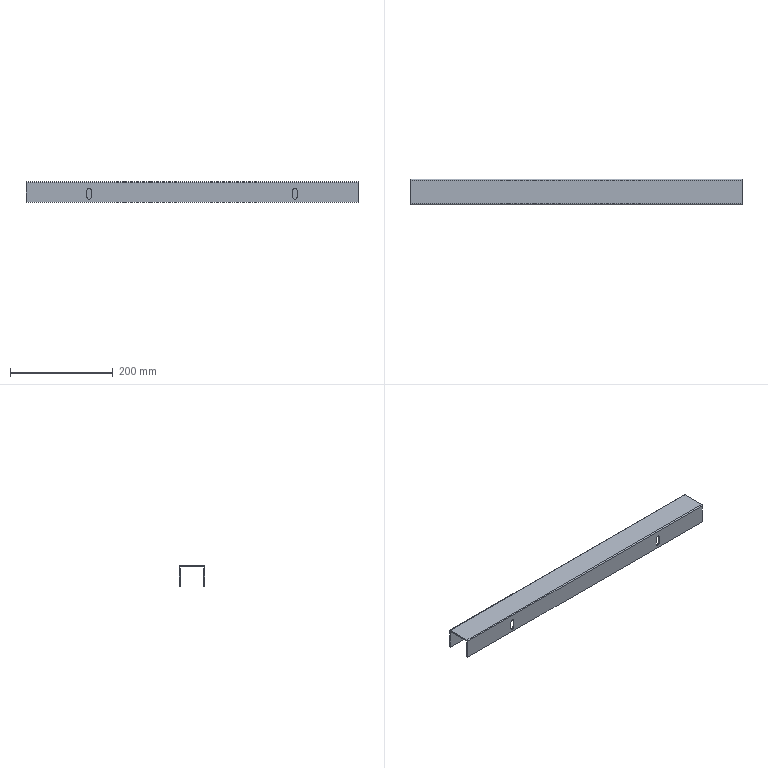Component | SolidWorks | FrameAssembly-1_FrameWeldment-1_FrontBendPlate-1 | 1 solid | 20 faces | box 645 x 50 x 40 mm | volume 199597 mm3 | plane 14 | cylinder 6 | commonest cylinder face diameters 9 x4 4 x2
STEP:
#1=COLOUR_RGB('',0.7922,0.8196,0.9333);
#2=FILL_AREA_STYLE_COLOUR('',#1);
#3=FILL_AREA_STYLE('',(#2));
#4=SURFACE_STYLE_FILL_AREA(#3);
#5=SURFACE_SIDE_STYLE('',(#4));
#6=SURFACE_STYLE_USAGE(.BOTH.,#5);
#7=PRESENTATION_STYLE_ASSIGNMENT((#6));
#8=CARTESIAN_POINT('',(-24.459,-6.068,13.327));
#9=VERTEX_POINT('',#8);
#10=CARTESIAN_POINT('',(0.9352,-6.068,13.327));
#11=VERTEX_POINT('',#10);
#12=CARTESIAN_POINT('',(-24.459,-6.068,13.327));
#13=DIRECTION('',(1.,-0.,-0.));
#14=VECTOR('',#13,39.37);
#15=LINE('',#12,#14);
#16=EDGE_CURVE('',#9,#11,#15,.T.);
#17=ORIENTED_EDGE('',*,*,#16,.T.);
#18=CARTESIAN_POINT('',(0.9352,-6.166,13.327));
#19=VERTEX_POINT('',#18);
#20=CARTESIAN_POINT('',(0.9352,-4.198,13.327));
#21=DIRECTION('',(-0.,-1.,0.));
#22=VECTOR('',#21,39.37);
#23=LINE('',#20,#22);
#24=EDGE_CURVE('',#11,#19,#23,.T.);
#25=ORIENTED_EDGE('',*,*,#24,.T.);
#26=CARTESIAN_POINT('',(-24.459,-6.166,13.327));
#27=VERTEX_POINT('',#26);
#28=CARTESIAN_POINT('',(0.9352,-6.166,13.327));
#29=DIRECTION('',(-1.,0.,0.));
#30=VECTOR('',#29,39.37);
#31=LINE('',#28,#30);
#32=EDGE_CURVE('',#19,#27,#31,.T.);
#33=ORIENTED_EDGE('',*,*,#32,.T.);
#34=CARTESIAN_POINT('',(-24.459,-4.198,13.327));
#35=DIRECTION('',(-0.,-1.,0.));
#36=VECTOR('',#35,39.37);
#37=LINE('',#34,#36);
#38=EDGE_CURVE('',#9,#27,#37,.T.);
#39=ORIENTED_EDGE('',*,*,#38,.F.);
#40=EDGE_LOOP('',(#17,#25,#33,#39));
#41=FACE_OUTER_BOUND('',#40,.T.);
#42=CARTESIAN_POINT('',(0.9352,-4.198,13.327));
#43=DIRECTION('',(-0.,-0.,-1.));
#44=DIRECTION('',(-1.,0.,0.));
#45=AXIS2_PLACEMENT_3D('',#42,#43,#44);
#46=PLANE('',#45);
#47=ADVANCED_FACE('',(#41),#46,.T.);
#48=CARTESIAN_POINT('',(-24.459,-4.198,14.823));
#49=VERTEX_POINT('',#48);
#50=CARTESIAN_POINT('',(-24.459,-4.198,13.327));
#51=VERTEX_POINT('',#50);
#52=CARTESIAN_POINT('',(-24.459,-4.198,14.823));
#53=DIRECTION('',(-0.,-0.,-1.));
#54=VECTOR('',#53,39.37);
#55=LINE('',#52,#54);
#56=EDGE_CURVE('',#49,#51,#55,.T.);
#57=ORIENTED_EDGE('',*,*,#56,.F.);
#58=CARTESIAN_POINT('',(0.9352,-4.198,14.823));
#59=VERTEX_POINT('',#58);
#60=CARTESIAN_POINT('',(0.9352,-4.198,14.823));
#61=DIRECTION('',(-1.,0.,0.));
#62=VECTOR('',#61,39.37);
#63=LINE('',#60,#62);
#64=EDGE_CURVE('',#59,#49,#63,.T.);
#65=ORIENTED_EDGE('',*,*,#64,.F.);
#66=CARTESIAN_POINT('',(0.9352,-4.198,13.327));
#67=VERTEX_POINT('',#66);
#68=CARTESIAN_POINT('',(0.9352,-4.198,14.823));
#69=DIRECTION('',(-0.,-0.,-1.));
#70=VECTOR('',#69,39.37);
#71=LINE('',#68,#70);
#72=EDGE_CURVE('',#59,#67,#71,.T.);
#73=ORIENTED_EDGE('',*,*,#72,.T.);
#74=CARTESIAN_POINT('',(0.9352,-4.198,13.327));
#75=DIRECTION('',(-1.,0.,0.));
#76=VECTOR('',#75,39.37);
#77=LINE('',#74,#76);
#78=EDGE_CURVE('',#67,#51,#77,.T.);
#79=ORIENTED_EDGE('',*,*,#78,.T.);
#80=EDGE_LOOP('',(#57,#65,#73,#79));
#81=FACE_OUTER_BOUND('',#80,.T.);
#82=CARTESIAN_POINT('',(0.9352,-4.198,14.823));
#83=DIRECTION('',(0.,1.,-0.));
#84=DIRECTION('',(1.,-0.,-0.));
#85=AXIS2_PLACEMENT_3D('',#82,#83,#84);
#86=PLANE('',#85);
#87=ADVANCED_FACE('',(#81),#86,.T.);
#88=CARTESIAN_POINT('',(-24.459,-4.277,14.902));
#89=VERTEX_POINT('',#88);
#90=CARTESIAN_POINT('',(-24.459,-4.277,14.823));
#91=DIRECTION('',(-1.,0.,0.));
#92=DIRECTION('',(0.,0.,1.));
#93=AXIS2_PLACEMENT_3D('',#90,#91,#92);
#94=CIRCLE('',#93,0.07874);
#95=EDGE_CURVE('',#89,#49,#94,.T.);
#96=ORIENTED_EDGE('',*,*,#95,.F.);
#97=CARTESIAN_POINT('',(0.9352,-4.277,14.902));
#98=VERTEX_POINT('',#97);
#99=CARTESIAN_POINT('',(0.9352,-4.277,14.902));
#100=DIRECTION('',(-1.,0.,0.));
#101=VECTOR('',#100,39.37);
#102=LINE('',#99,#101);
#103=EDGE_CURVE('',#98,#89,#102,.T.);
#104=ORIENTED_EDGE('',*,*,#103,.F.);
#105=CARTESIAN_POINT('',(0.9352,-4.277,14.823));
#106=DIRECTION('',(-1.,0.,0.));
#107=DIRECTION('',(0.,0.,1.));
#108=AXIS2_PLACEMENT_3D('',#105,#106,#107);
#109=CIRCLE('',#108,0.07874);
#110=EDGE_CURVE('',#98,#59,#109,.T.);
#111=ORIENTED_EDGE('',*,*,#110,.T.);
#112=ORIENTED_EDGE('',*,*,#64,.T.);
#113=EDGE_LOOP('',(#96,#104,#111,#112));
#114=FACE_OUTER_BOUND('',#113,.T.);
#115=CARTESIAN_POINT('',(0.9352,-4.277,14.823));
#116=DIRECTION('',(-1.,0.,0.));
#117=DIRECTION('',(0.,0.,1.));
#118=AXIS2_PLACEMENT_3D('',#115,#116,#117);
#119=CYLINDRICAL_SURFACE('',#118,0.07874);
#120=ADVANCED_FACE('',(#114),#119,.T.);
#121=CARTESIAN_POINT('',(-24.459,-6.088,14.902));
#122=VERTEX_POINT('',#121);
#123=CARTESIAN_POINT('',(-24.459,-6.088,14.902));
#124=DIRECTION('',(0.,1.,0.));
#125=VECTOR('',#124,39.37);
#126=LINE('',#123,#125);
#127=EDGE_CURVE('',#122,#89,#126,.T.);
#128=ORIENTED_EDGE('',*,*,#127,.F.);
#129=CARTESIAN_POINT('',(0.9352,-6.088,14.902));
#130=VERTEX_POINT('',#129);
#131=CARTESIAN_POINT('',(0.9352,-6.088,14.902));
#132=DIRECTION('',(-1.,0.,0.));
#133=VECTOR('',#132,39.37);
#134=LINE('',#131,#133);
#135=EDGE_CURVE('',#130,#122,#134,.T.);
#136=ORIENTED_EDGE('',*,*,#135,.F.);
#137=CARTESIAN_POINT('',(0.9352,-6.088,14.902));
#138=DIRECTION('',(0.,1.,0.));
#139=VECTOR('',#138,39.37);
#140=LINE('',#137,#139);
#141=EDGE_CURVE('',#130,#98,#140,.T.);
#142=ORIENTED_EDGE('',*,*,#141,.T.);
#143=ORIENTED_EDGE('',*,*,#103,.T.);
#144=EDGE_LOOP('',(#128,#136,#142,#143));
#145=FACE_OUTER_BOUND('',#144,.T.);
#146=CARTESIAN_POINT('',(0.9352,-6.088,14.902));
#147=DIRECTION('',(0.,-0.,1.));
#148=DIRECTION('',(-0.,-1.,-0.));
#149=AXIS2_PLACEMENT_3D('',#146,#147,#148);
#150=PLANE('',#149);
#151=ADVANCED_FACE('',(#145),#150,.T.);
#152=CARTESIAN_POINT('',(-24.459,-6.166,14.823));
#153=VERTEX_POINT('',#152);
#154=CARTESIAN_POINT('',(-24.459,-6.088,14.823));
#155=DIRECTION('',(-1.,0.,0.));
#156=DIRECTION('',(0.,0.,1.));
#157=AXIS2_PLACEMENT_3D('',#154,#155,#156);
#158=CIRCLE('',#157,0.07874);
#159=EDGE_CURVE('',#153,#122,#158,.T.);
#160=ORIENTED_EDGE('',*,*,#159,.F.);
#161=CARTESIAN_POINT('',(0.9352,-6.166,14.823));
#162=VERTEX_POINT('',#161);
#163=CARTESIAN_POINT('',(0.9352,-6.166,14.823));
#164=DIRECTION('',(-1.,0.,0.));
#165=VECTOR('',#164,39.37);
#166=LINE('',#163,#165);
#167=EDGE_CURVE('',#162,#153,#166,.T.);
#168=ORIENTED_EDGE('',*,*,#167,.F.);
#169=CARTESIAN_POINT('',(0.9352,-6.088,14.823));
#170=DIRECTION('',(-1.,0.,0.));
#171=DIRECTION('',(0.,0.,1.));
#172=AXIS2_PLACEMENT_3D('',#169,#170,#171);
#173=CIRCLE('',#172,0.07874);
#174=EDGE_CURVE('',#162,#130,#173,.T.);
#175=ORIENTED_EDGE('',*,*,#174,.T.);
#176=ORIENTED_EDGE('',*,*,#135,.T.);
#177=EDGE_LOOP('',(#160,#168,#175,#176));
#178=FACE_OUTER_BOUND('',#177,.T.);
#179=CARTESIAN_POINT('',(0.9352,-6.088,14.823));
#180=DIRECTION('',(-1.,0.,0.));
#181=DIRECTION('',(0.,0.,1.));
#182=AXIS2_PLACEMENT_3D('',#179,#180,#181);
#183=CYLINDRICAL_SURFACE('',#182,0.07874);
#184=ADVANCED_FACE('',(#178),#183,.T.);
#185=CARTESIAN_POINT('',(-19.813,-6.166,13.74));
#186=VERTEX_POINT('',#185);
#187=CARTESIAN_POINT('',(-19.459,-6.166,13.74));
#188=VERTEX_POINT('',#187);
#189=CARTESIAN_POINT('',(-19.636,-6.166,13.74));
#190=DIRECTION('',(-0.,-1.,0.));
#191=DIRECTION('',(-1.,0.,0.));
#192=AXIS2_PLACEMENT_3D('',#189,#190,#191);
#193=CIRCLE('',#192,0.1772);
#194=EDGE_CURVE('',#186,#188,#193,.T.);
#195=ORIENTED_EDGE('',*,*,#194,.F.);
#196=CARTESIAN_POINT('',(-19.813,-6.166,14.213));
#197=VERTEX_POINT('',#196);
#198=CARTESIAN_POINT('',(-19.813,-6.166,14.213));
#199=DIRECTION('',(-0.,-0.,-1.));
#200=VECTOR('',#199,39.37);
#201=LINE('',#198,#200);
#202=EDGE_CURVE('',#197,#186,#201,.T.);
#203=ORIENTED_EDGE('',*,*,#202,.F.);
#204=CARTESIAN_POINT('',(-19.459,-6.166,14.213));
#205=VERTEX_POINT('',#204);
#206=CARTESIAN_POINT('',(-19.636,-6.166,14.213));
#207=DIRECTION('',(-0.,-1.,0.));
#208=DIRECTION('',(-1.,0.,0.));
#209=AXIS2_PLACEMENT_3D('',#206,#207,#208);
#210=CIRCLE('',#209,0.1772);
#211=EDGE_CURVE('',#205,#197,#210,.T.);
#212=ORIENTED_EDGE('',*,*,#211,.F.);
#213=CARTESIAN_POINT('',(-19.459,-6.166,13.74));
#214=DIRECTION('',(0.,0.,1.));
#215=VECTOR('',#214,39.37);
#216=LINE('',#213,#215);
#217=EDGE_CURVE('',#188,#205,#216,.T.);
#218=ORIENTED_EDGE('',*,*,#217,.F.);
#219=EDGE_LOOP('',(#195,#203,#212,#218));
#220=FACE_BOUND('',#219,.T.);
#221=CARTESIAN_POINT('',(-3.71,-6.166,13.74));
#222=VERTEX_POINT('',#221);
#223=CARTESIAN_POINT('',(-4.065,-6.166,13.74));
#224=VERTEX_POINT('',#223);
#225=CARTESIAN_POINT('',(-3.888,-6.166,13.74));
#226=DIRECTION('',(0.,1.,-0.));
#227=DIRECTION('',(1.,0.,0.));
#228=AXIS2_PLACEMENT_3D('',#225,#226,#227);
#229=CIRCLE('',#228,0.1772);
#230=EDGE_CURVE('',#222,#224,#229,.T.);
#231=ORIENTED_EDGE('',*,*,#230,.T.);
#232=CARTESIAN_POINT('',(-4.065,-6.166,14.213));
#233=VERTEX_POINT('',#232);
#234=CARTESIAN_POINT('',(-4.065,-6.166,13.74));
#235=DIRECTION('',(0.,0.,1.));
#236=VECTOR('',#235,39.37);
#237=LINE('',#234,#236);
#238=EDGE_CURVE('',#224,#233,#237,.T.);
#239=ORIENTED_EDGE('',*,*,#238,.T.);
#240=CARTESIAN_POINT('',(-3.71,-6.166,14.213));
#241=VERTEX_POINT('',#240);
#242=CARTESIAN_POINT('',(-3.888,-6.166,14.213));
#243=DIRECTION('',(0.,1.,-0.));
#244=DIRECTION('',(1.,0.,0.));
#245=AXIS2_PLACEMENT_3D('',#242,#243,#244);
#246=CIRCLE('',#245,0.1772);
#247=EDGE_CURVE('',#233,#241,#246,.T.);
#248=ORIENTED_EDGE('',*,*,#247,.T.);
#249=CARTESIAN_POINT('',(-3.71,-6.166,14.213));
#250=DIRECTION('',(-0.,-0.,-1.));
#251=VECTOR('',#250,39.37);
#252=LINE('',#249,#251);
#253=EDGE_CURVE('',#241,#222,#252,.T.);
#254=ORIENTED_EDGE('',*,*,#253,.T.);
#255=EDGE_LOOP('',(#231,#239,#248,#254));
#256=FACE_BOUND('',#255,.T.);
#257=CARTESIAN_POINT('',(-24.459,-6.166,13.327));
#258=DIRECTION('',(0.,0.,1.));
#259=VECTOR('',#258,39.37);
#260=LINE('',#257,#259);
#261=EDGE_CURVE('',#27,#153,#260,.T.);
#262=ORIENTED_EDGE('',*,*,#261,.F.);
#263=ORIENTED_EDGE('',*,*,#32,.F.);
#264=CARTESIAN_POINT('',(0.9352,-6.166,13.327));
#265=DIRECTION('',(0.,0.,1.));
#266=VECTOR('',#265,39.37);
#267=LINE('',#264,#266);
#268=EDGE_CURVE('',#19,#162,#267,.T.);
#269=ORIENTED_EDGE('',*,*,#268,.T.);
#270=ORIENTED_EDGE('',*,*,#167,.T.);
#271=EDGE_LOOP('',(#262,#263,#269,#270));
#272=FACE_OUTER_BOUND('',#271,.T.);
#273=CARTESIAN_POINT('',(0.9352,-6.166,13.327));
#274=DIRECTION('',(-0.,-1.,0.));
#275=DIRECTION('',(-1.,0.,0.));
#276=AXIS2_PLACEMENT_3D('',#273,#274,#275);
#277=PLANE('',#276);
#278=ADVANCED_FACE('',(#220,#256,#272),#277,.T.);
#279=CARTESIAN_POINT('',(-24.459,-4.296,13.327));
#280=VERTEX_POINT('',#279);
#281=CARTESIAN_POINT('',(0.9352,-4.296,13.327));
#282=VERTEX_POINT('',#281);
#283=CARTESIAN_POINT('',(-24.459,-4.296,13.327));
#284=DIRECTION('',(1.,-0.,-0.));
#285=VECTOR('',#284,39.37);
#286=LINE('',#283,#285);
#287=EDGE_CURVE('',#280,#282,#286,.T.);
#288=ORIENTED_EDGE('',*,*,#287,.F.);
#289=CARTESIAN_POINT('',(-24.459,-4.198,13.327));
#290=DIRECTION('',(-0.,-1.,0.));
#291=VECTOR('',#290,39.37);
#292=LINE('',#289,#291);
#293=EDGE_CURVE('',#51,#280,#292,.T.);
#294=ORIENTED_EDGE('',*,*,#293,.F.);
#295=ORIENTED_EDGE('',*,*,#78,.F.);
#296=CARTESIAN_POINT('',(0.9352,-4.198,13.327));
#297=DIRECTION('',(-0.,-1.,0.));
#298=VECTOR('',#297,39.37);
#299=LINE('',#296,#298);
#300=EDGE_CURVE('',#67,#282,#299,.T.);
#301=ORIENTED_EDGE('',*,*,#300,.T.);
#302=EDGE_LOOP('',(#288,#294,#295,#301));
#303=FACE_OUTER_BOUND('',#302,.T.);
#304=CARTESIAN_POINT('',(0.9352,-4.198,13.327));
#305=DIRECTION('',(-0.,-0.,-1.));
#306=DIRECTION('',(-1.,0.,0.));
#307=AXIS2_PLACEMENT_3D('',#304,#305,#306);
#308=PLANE('',#307);
#309=ADVANCED_FACE('',(#303),#308,.T.);
#310=ORIENTED_EDGE('',*,*,#24,.F.);
#311=CARTESIAN_POINT('',(0.9352,-6.068,14.803));
#312=VERTEX_POINT('',#311);
#313=CARTESIAN_POINT('',(0.9352,-6.068,14.803));
#314=DIRECTION('',(-0.,-0.,-1.));
#315=VECTOR('',#314,39.37);
#316=LINE('',#313,#315);
#317=EDGE_CURVE('',#312,#11,#316,.T.);
#318=ORIENTED_EDGE('',*,*,#317,.F.);
#319=CARTESIAN_POINT('',(0.9352,-4.296,14.803));
#320=VERTEX_POINT('',#319);
#321=CARTESIAN_POINT('',(0.9352,-4.296,14.803));
#322=DIRECTION('',(-0.,-1.,0.));
#323=VECTOR('',#322,39.37);
#324=LINE('',#321,#323);
#325=EDGE_CURVE('',#320,#312,#324,.T.);
#326=ORIENTED_EDGE('',*,*,#325,.F.);
#327=CARTESIAN_POINT('',(0.9352,-4.296,13.327));
#328=DIRECTION('',(0.,0.,1.));
#329=VECTOR('',#328,39.37);
#330=LINE('',#327,#329);
#331=EDGE_CURVE('',#282,#320,#330,.T.);
#332=ORIENTED_EDGE('',*,*,#331,.F.);
#333=ORIENTED_EDGE('',*,*,#300,.F.);
#334=ORIENTED_EDGE('',*,*,#72,.F.);
#335=ORIENTED_EDGE('',*,*,#110,.F.);
#336=ORIENTED_EDGE('',*,*,#141,.F.);
#337=ORIENTED_EDGE('',*,*,#174,.F.);
#338=ORIENTED_EDGE('',*,*,#268,.F.);
#339=EDGE_LOOP('',(#310,#318,#326,#332,#333,#334,#335,#336,#337,#338));
#340=FACE_OUTER_BOUND('',#339,.T.);
#341=CARTESIAN_POINT('',(0.9352,-6.088,14.823));
#342=DIRECTION('',(-1.,0.,0.));
#343=DIRECTION('',(0.,0.,1.));
#344=AXIS2_PLACEMENT_3D('',#341,#342,#343);
#345=PLANE('',#344);
#346=ADVANCED_FACE('',(#340),#345,.F.);
#347=CARTESIAN_POINT('',(-24.459,-6.068,14.803));
#348=VERTEX_POINT('',#347);
#349=CARTESIAN_POINT('',(-24.459,-6.068,14.803));
#350=DIRECTION('',(-0.,-0.,-1.));
#351=VECTOR('',#350,39.37);
#352=LINE('',#349,#351);
#353=EDGE_CURVE('',#348,#9,#352,.T.);
#354=ORIENTED_EDGE('',*,*,#353,.T.);
#355=ORIENTED_EDGE('',*,*,#38,.T.);
#356=ORIENTED_EDGE('',*,*,#261,.T.);
#357=ORIENTED_EDGE('',*,*,#159,.T.);
#358=ORIENTED_EDGE('',*,*,#127,.T.);
#359=ORIENTED_EDGE('',*,*,#95,.T.);
#360=ORIENTED_EDGE('',*,*,#56,.T.);
#361=ORIENTED_EDGE('',*,*,#293,.T.);
#362=CARTESIAN_POINT('',(-24.459,-4.296,14.803));
#363=VERTEX_POINT('',#362);
#364=CARTESIAN_POINT('',(-24.459,-4.296,13.327));
#365=DIRECTION('',(0.,0.,1.));
#366=VECTOR('',#365,39.37);
#367=LINE('',#364,#366);
#368=EDGE_CURVE('',#280,#363,#367,.T.);
#369=ORIENTED_EDGE('',*,*,#368,.T.);
#370=CARTESIAN_POINT('',(-24.459,-4.296,14.803));
#371=DIRECTION('',(-0.,-1.,0.));
#372=VECTOR('',#371,39.37);
#373=LINE('',#370,#372);
#374=EDGE_CURVE('',#363,#348,#373,.T.);
#375=ORIENTED_EDGE('',*,*,#374,.T.);
#376=EDGE_LOOP('',(#354,#355,#356,#357,#358,#359,#360,#361,#369,#375));
#377=FACE_OUTER_BOUND('',#376,.T.);
#378=CARTESIAN_POINT('',(-24.459,-6.088,14.823));
#379=DIRECTION('',(-1.,0.,0.));
#380=DIRECTION('',(0.,0.,1.));
#381=AXIS2_PLACEMENT_3D('',#378,#379,#380);
#382=PLANE('',#381);
#383=ADVANCED_FACE('',(#377),#382,.T.);
#384=CARTESIAN_POINT('',(-19.813,-6.068,13.74));
#385=VERTEX_POINT('',#384);
#386=CARTESIAN_POINT('',(-19.813,-6.068,14.213));
#387=VERTEX_POINT('',#386);
#388=CARTESIAN_POINT('',(-19.813,-6.068,14.213));
#389=DIRECTION('',(0.,0.,1.));
#390=VECTOR('',#389,39.37);
#391=LINE('',#388,#390);
#392=EDGE_CURVE('',#385,#387,#391,.T.);
#393=ORIENTED_EDGE('',*,*,#392,.F.);
#394=CARTESIAN_POINT('',(-19.459,-6.068,13.74));
#395=VERTEX_POINT('',#394);
#396=CARTESIAN_POINT('',(-19.636,-6.068,13.74));
#397=DIRECTION('',(0.,1.,-0.));
#398=DIRECTION('',(-1.,0.,0.));
#399=AXIS2_PLACEMENT_3D('',#396,#397,#398);
#400=CIRCLE('',#399,0.1772);
#401=EDGE_CURVE('',#395,#385,#400,.T.);
#402=ORIENTED_EDGE('',*,*,#401,.F.);
#403=CARTESIAN_POINT('',(-19.459,-6.068,14.213));
#404=VERTEX_POINT('',#403);
#405=CARTESIAN_POINT('',(-19.459,-6.068,13.74));
#406=DIRECTION('',(-0.,-0.,-1.));
#407=VECTOR('',#406,39.37);
#408=LINE('',#405,#407);
#409=EDGE_CURVE('',#404,#395,#408,.T.);
#410=ORIENTED_EDGE('',*,*,#409,.F.);
#411=CARTESIAN_POINT('',(-19.636,-6.068,14.213));
#412=DIRECTION('',(0.,1.,-0.));
#413=DIRECTION('',(-1.,0.,0.));
#414=AXIS2_PLACEMENT_3D('',#411,#412,#413);
#415=CIRCLE('',#414,0.1772);
#416=EDGE_CURVE('',#387,#404,#415,.T.);
#417=ORIENTED_EDGE('',*,*,#416,.F.);
#418=EDGE_LOOP('',(#393,#402,#410,#417));
#419=FACE_BOUND('',#418,.T.);
#420=CARTESIAN_POINT('',(-4.065,-6.068,13.74));
#421=VERTEX_POINT('',#420);
#422=CARTESIAN_POINT('',(-4.065,-6.068,14.213));
#423=VERTEX_POINT('',#422);
#424=CARTESIAN_POINT('',(-4.065,-6.068,13.74));
#425=DIRECTION('',(0.,0.,1.));
#426=VECTOR('',#425,39.37);
#427=LINE('',#424,#426);
#428=EDGE_CURVE('',#421,#423,#427,.T.);
#429=ORIENTED_EDGE('',*,*,#428,.F.);
#430=CARTESIAN_POINT('',(-3.71,-6.068,13.74));
#431=VERTEX_POINT('',#430);
#432=CARTESIAN_POINT('',(-3.888,-6.068,13.74));
#433=DIRECTION('',(0.,1.,-0.));
#434=DIRECTION('',(1.,0.,0.));
#435=AXIS2_PLACEMENT_3D('',#432,#433,#434);
#436=CIRCLE('',#435,0.1772);
#437=EDGE_CURVE('',#431,#421,#436,.T.);
#438=ORIENTED_EDGE('',*,*,#437,.F.);
#439=CARTESIAN_POINT('',(-3.71,-6.068,14.213));
#440=VERTEX_POINT('',#439);
#441=CARTESIAN_POINT('',(-3.71,-6.068,14.213));
#442=DIRECTION('',(-0.,-0.,-1.));
#443=VECTOR('',#442,39.37);
#444=LINE('',#441,#443);
#445=EDGE_CURVE('',#440,#431,#444,.T.);
#446=ORIENTED_EDGE('',*,*,#445,.F.);
#447=CARTESIAN_POINT('',(-3.888,-6.068,14.213));
#448=DIRECTION('',(0.,1.,-0.));
#449=DIRECTION('',(1.,0.,0.));
#450=AXIS2_PLACEMENT_3D('',#447,#448,#449);
#451=CIRCLE('',#450,0.1772);
#452=EDGE_CURVE('',#423,#440,#451,.T.);
#453=ORIENTED_EDGE('',*,*,#452,.F.);
#454=EDGE_LOOP('',(#429,#438,#446,#453));
#455=FACE_BOUND('',#454,.T.);
#456=ORIENTED_EDGE('',*,*,#317,.T.);
#457=ORIENTED_EDGE('',*,*,#16,.F.);
#458=ORIENTED_EDGE('',*,*,#353,.F.);
#459=CARTESIAN_POINT('',(-24.459,-6.068,14.803));
#460=DIRECTION('',(1.,-0.,-0.));
#461=VECTOR('',#460,39.37);
#462=LINE('',#459,#461);
#463=EDGE_CURVE('',#348,#312,#462,.T.);
#464=ORIENTED_EDGE('',*,*,#463,.T.);
#465=EDGE_LOOP('',(#456,#457,#458,#464));
#466=FACE_OUTER_BOUND('',#465,.T.);
#467=CARTESIAN_POINT('',(-24.459,-6.068,14.803));
#468=DIRECTION('',(-0.,-1.,0.));
#469=DIRECTION('',(-1.,0.,0.));
#470=AXIS2_PLACEMENT_3D('',#467,#468,#469);
#471=PLANE('',#470);
#472=ADVANCED_FACE('',(#419,#455,#466),#471,.F.);
#473=ORIENTED_EDGE('',*,*,#325,.T.);
#474=ORIENTED_EDGE('',*,*,#463,.F.);
#475=ORIENTED_EDGE('',*,*,#374,.F.);
#476=CARTESIAN_POINT('',(-24.459,-4.296,14.803));
#477=DIRECTION('',(1.,-0.,-0.));
#478=VECTOR('',#477,39.37);
#479=LINE('',#476,#478);
#480=EDGE_CURVE('',#363,#320,#479,.T.);
#481=ORIENTED_EDGE('',*,*,#480,.T.);
#482=EDGE_LOOP('',(#473,#474,#475,#481));
#483=FACE_OUTER_BOUND('',#482,.T.);
#484=CARTESIAN_POINT('',(-24.459,-4.296,14.803));
#485=DIRECTION('',(0.,0.,1.));
#486=DIRECTION('',(1.,-0.,-0.));
#487=AXIS2_PLACEMENT_3D('',#484,#485,#486);
#488=PLANE('',#487);
#489=ADVANCED_FACE('',(#483),#488,.F.);
#490=ORIENTED_EDGE('',*,*,#331,.T.);
#491=ORIENTED_EDGE('',*,*,#480,.F.);
#492=ORIENTED_EDGE('',*,*,#368,.F.);
#493=ORIENTED_EDGE('',*,*,#287,.T.);
#494=EDGE_LOOP('',(#490,#491,#492,#493));
#495=FACE_OUTER_BOUND('',#494,.T.);
#496=CARTESIAN_POINT('',(-24.459,-4.296,13.327));
#497=DIRECTION('',(0.,1.,-0.));
#498=DIRECTION('',(1.,-0.,-0.));
#499=AXIS2_PLACEMENT_3D('',#496,#497,#498);
#500=PLANE('',#499);
#501=ADVANCED_FACE('',(#495),#500,.F.);
#502=ORIENTED_EDGE('',*,*,#437,.T.);
#503=CARTESIAN_POINT('',(-4.065,-6.166,13.74));
#504=DIRECTION('',(0.,1.,-0.));
#505=VECTOR('',#504,39.37);
#506=LINE('',#503,#505);
#507=EDGE_CURVE('',#224,#421,#506,.T.);
#508=ORIENTED_EDGE('',*,*,#507,.F.);
#509=ORIENTED_EDGE('',*,*,#230,.F.);
#510=CARTESIAN_POINT('',(-3.71,-6.166,13.74));
#511=DIRECTION('',(0.,1.,-0.));
#512=VECTOR('',#511,39.37);
#513=LINE('',#510,#512);
#514=EDGE_CURVE('',#222,#431,#513,.T.);
#515=ORIENTED_EDGE('',*,*,#514,.T.);
#516=EDGE_LOOP('',(#502,#508,#509,#515));
#517=FACE_OUTER_BOUND('',#516,.T.);
#518=CARTESIAN_POINT('',(-3.888,-6.166,13.74));
#519=DIRECTION('',(0.,1.,-0.));
#520=DIRECTION('',(1.,0.,0.));
#521=AXIS2_PLACEMENT_3D('',#518,#519,#520);
#522=CYLINDRICAL_SURFACE('',#521,0.1772);
#523=ADVANCED_FACE('',(#517),#522,.F.);
#524=ORIENTED_EDGE('',*,*,#445,.T.);
#525=ORIENTED_EDGE('',*,*,#514,.F.);
#526=ORIENTED_EDGE('',*,*,#253,.F.);
#527=CARTESIAN_POINT('',(-3.71,-6.166,14.213));
#528=DIRECTION('',(0.,1.,-0.));
#529=VECTOR('',#528,39.37);
#530=LINE('',#527,#529);
#531=EDGE_CURVE('',#241,#440,#530,.T.);
#532=ORIENTED_EDGE('',*,*,#531,.T.);
#533=EDGE_LOOP('',(#524,#525,#526,#532));
#534=FACE_OUTER_BOUND('',#533,.T.);
#535=CARTESIAN_POINT('',(-3.71,-6.166,14.213));
#536=DIRECTION('',(1.,-0.,-0.));
#537=DIRECTION('',(-0.,-0.,-1.));
#538=AXIS2_PLACEMENT_3D('',#535,#536,#537);
#539=PLANE('',#538);
#540=ADVANCED_FACE('',(#534),#539,.F.);
#541=ORIENTED_EDGE('',*,*,#452,.T.);
#542=ORIENTED_EDGE('',*,*,#531,.F.);
#543=ORIENTED_EDGE('',*,*,#247,.F.);
#544=CARTESIAN_POINT('',(-4.065,-6.166,14.213));
#545=DIRECTION('',(0.,1.,-0.));
#546=VECTOR('',#545,39.37);
#547=LINE('',#544,#546);
#548=EDGE_CURVE('',#233,#423,#547,.T.);
#549=ORIENTED_EDGE('',*,*,#548,.T.);
#550=EDGE_LOOP('',(#541,#542,#543,#549));
#551=FACE_OUTER_BOUND('',#550,.T.);
#552=CARTESIAN_POINT('',(-3.888,-6.166,14.213));
#553=DIRECTION('',(0.,1.,-0.));
#554=DIRECTION('',(1.,0.,0.));
#555=AXIS2_PLACEMENT_3D('',#552,#553,#554);
#556=CYLINDRICAL_SURFACE('',#555,0.1772);
#557=ADVANCED_FACE('',(#551),#556,.F.);
#558=ORIENTED_EDGE('',*,*,#428,.T.);
#559=ORIENTED_EDGE('',*,*,#548,.F.);
#560=ORIENTED_EDGE('',*,*,#238,.F.);
#561=ORIENTED_EDGE('',*,*,#507,.T.);
#562=EDGE_LOOP('',(#558,#559,#560,#561));
#563=FACE_OUTER_BOUND('',#562,.T.);
#564=CARTESIAN_POINT('',(-4.065,-6.166,13.74));
#565=DIRECTION('',(-1.,0.,0.));
#566=DIRECTION('',(0.,0.,1.));
#567=AXIS2_PLACEMENT_3D('',#564,#565,#566);
#568=PLANE('',#567);
#569=ADVANCED_FACE('',(#563),#568,.F.);
#570=ORIENTED_EDGE('',*,*,#401,.T.);
#571=CARTESIAN_POINT('',(-19.813,-4.198,13.74));
#572=DIRECTION('',(-0.,-1.,0.));
#573=VECTOR('',#572,39.37);
#574=LINE('',#571,#573);
#575=EDGE_CURVE('',#385,#186,#574,.T.);
#576=ORIENTED_EDGE('',*,*,#575,.T.);
#577=ORIENTED_EDGE('',*,*,#194,.T.);
#578=CARTESIAN_POINT('',(-19.459,-4.198,13.74));
#579=DIRECTION('',(-0.,-1.,0.));
#580=VECTOR('',#579,39.37);
#581=LINE('',#578,#580);
#582=EDGE_CURVE('',#395,#188,#581,.T.);
#583=ORIENTED_EDGE('',*,*,#582,.F.);
#584=EDGE_LOOP('',(#570,#576,#577,#583));
#585=FACE_OUTER_BOUND('',#584,.T.);
#586=CARTESIAN_POINT('',(-19.636,-4.198,13.74));
#587=DIRECTION('',(-0.,-1.,0.));
#588=DIRECTION('',(-1.,0.,0.));
#589=AXIS2_PLACEMENT_3D('',#586,#587,#588);
#590=CYLINDRICAL_SURFACE('',#589,0.1772);
#591=ADVANCED_FACE('',(#585),#590,.F.);
#592=ORIENTED_EDGE('',*,*,#392,.T.);
#593=CARTESIAN_POINT('',(-19.813,-4.198,14.213));
#594=DIRECTION('',(-0.,-1.,0.));
#595=VECTOR('',#594,39.37);
#596=LINE('',#593,#595);
#597=EDGE_CURVE('',#387,#197,#596,.T.);
#598=ORIENTED_EDGE('',*,*,#597,.T.);
#599=ORIENTED_EDGE('',*,*,#202,.T.);
#600=ORIENTED_EDGE('',*,*,#575,.F.);
#601=EDGE_LOOP('',(#592,#598,#599,#600));
#602=FACE_OUTER_BOUND('',#601,.T.);
#603=CARTESIAN_POINT('',(-19.813,-4.198,14.213));
#604=DIRECTION('',(-1.,0.,0.));
#605=DIRECTION('',(0.,0.,1.));
#606=AXIS2_PLACEMENT_3D('',#603,#604,#605);
#607=PLANE('',#606);
#608=ADVANCED_FACE('',(#602),#607,.F.);
#609=ORIENTED_EDGE('',*,*,#416,.T.);
#610=CARTESIAN_POINT('',(-19.459,-4.198,14.213));
#611=DIRECTION('',(-0.,-1.,0.));
#612=VECTOR('',#611,39.37);
#613=LINE('',#610,#612);
#614=EDGE_CURVE('',#404,#205,#613,.T.);
#615=ORIENTED_EDGE('',*,*,#614,.T.);
#616=ORIENTED_EDGE('',*,*,#211,.T.);
#617=ORIENTED_EDGE('',*,*,#597,.F.);
#618=EDGE_LOOP('',(#609,#615,#616,#617));
#619=FACE_OUTER_BOUND('',#618,.T.);
#620=CARTESIAN_POINT('',(-19.636,-4.198,14.213));
#621=DIRECTION('',(-0.,-1.,0.));
#622=DIRECTION('',(-1.,0.,0.));
#623=AXIS2_PLACEMENT_3D('',#620,#621,#622);
#624=CYLINDRICAL_SURFACE('',#623,0.1772);
#625=ADVANCED_FACE('',(#619),#624,.F.);
#626=ORIENTED_EDGE('',*,*,#409,.T.);
#627=ORIENTED_EDGE('',*,*,#582,.T.);
#628=ORIENTED_EDGE('',*,*,#217,.T.);
#629=ORIENTED_EDGE('',*,*,#614,.F.);
#630=EDGE_LOOP('',(#626,#627,#628,#629));
#631=FACE_OUTER_BOUND('',#630,.T.);
#632=CARTESIAN_POINT('',(-19.459,-4.198,13.74));
#633=DIRECTION('',(1.,-0.,-0.));
#634=DIRECTION('',(-0.,-0.,-1.));
#635=AXIS2_PLACEMENT_3D('',#632,#633,#634);
#636=PLANE('',#635);
#637=ADVANCED_FACE('',(#631),#636,.F.);
#638=CLOSED_SHELL('',(#47,#87,#120,#151,#184,#278,#309,#346,#383,#472,#489,#501,#523,#540,#557,#569,#591,#608,#625,#637));
#639=MANIFOLD_SOLID_BREP('',#638);
#640=STYLED_ITEM('',(#7),#639);
#641=(LENGTH_UNIT()NAMED_UNIT(*)SI_UNIT($,.METRE.));
#642=LENGTH_MEASURE_WITH_UNIT(LENGTH_MEASURE(0.0254),#641);
#643=DIMENSIONAL_EXPONENTS(1.,0.,0.,0.,0.,0.,0.);
#644=(CONVERSION_BASED_UNIT('',#642)LENGTH_UNIT()NAMED_UNIT(#643));
#645=UNCERTAINTY_MEASURE_WITH_UNIT(LENGTH_MEASURE(0.00001),#644,'','');
#646=(NAMED_UNIT(*)PLANE_ANGLE_UNIT()SI_UNIT($,.RADIAN.));
#647=(NAMED_UNIT(*)SI_UNIT($,.STERADIAN.)SOLID_ANGLE_UNIT());
#648=(GEOMETRIC_REPRESENTATION_CONTEXT(3)GLOBAL_UNCERTAINTY_ASSIGNED_CONTEXT((#645))GLOBAL_UNIT_ASSIGNED_CONTEXT((#644,#646,#647))REPRESENTATION_CONTEXT('',''));
#649=MECHANICAL_DESIGN_GEOMETRIC_PRESENTATION_REPRESENTATION('',(#640),#648);
#650=PRESENTATION_LAYER_ASSIGNMENT('','',(#640));
#651=CARTESIAN_POINT('',(0.,0.,0.));
#652=DIRECTION('',(0.,0.,1.));
#653=DIRECTION('',(1.,0.,0.));
#654=AXIS2_PLACEMENT_3D('',#651,#652,#653);
#655=(LENGTH_UNIT()NAMED_UNIT(*)SI_UNIT($,.METRE.));
#656=LENGTH_MEASURE_WITH_UNIT(LENGTH_MEASURE(0.0254),#655);
#657=DIMENSIONAL_EXPONENTS(1.,0.,0.,0.,0.,0.,0.);
#658=(CONVERSION_BASED_UNIT('',#656)LENGTH_UNIT()NAMED_UNIT(#657));
#659=UNCERTAINTY_MEASURE_WITH_UNIT(LENGTH_MEASURE(0.00001),#658,'','');
#660=(NAMED_UNIT(*)PLANE_ANGLE_UNIT()SI_UNIT($,.RADIAN.));
#661=(NAMED_UNIT(*)SI_UNIT($,.STERADIAN.)SOLID_ANGLE_UNIT());
#662=(GEOMETRIC_REPRESENTATION_CONTEXT(3)GLOBAL_UNCERTAINTY_ASSIGNED_CONTEXT((#659))GLOBAL_UNIT_ASSIGNED_CONTEXT((#658,#660,#661))REPRESENTATION_CONTEXT('',''));
#663=ADVANCED_BREP_SHAPE_REPRESENTATION('',(#639,#654),#662);